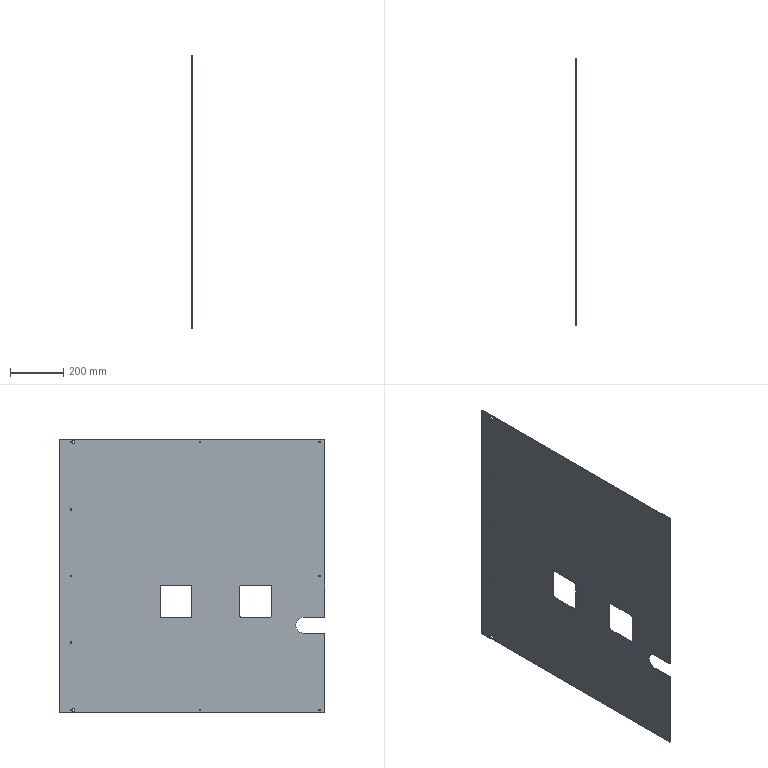Component | SolidWorks | SYM0671-81-105-2 | 1 solid | 54 faces | volume 1193418 mm3 | cylinder 33 | plane 21 | commonest cylinder face diameters 6 x18 10 x8 12 x6 60 x1